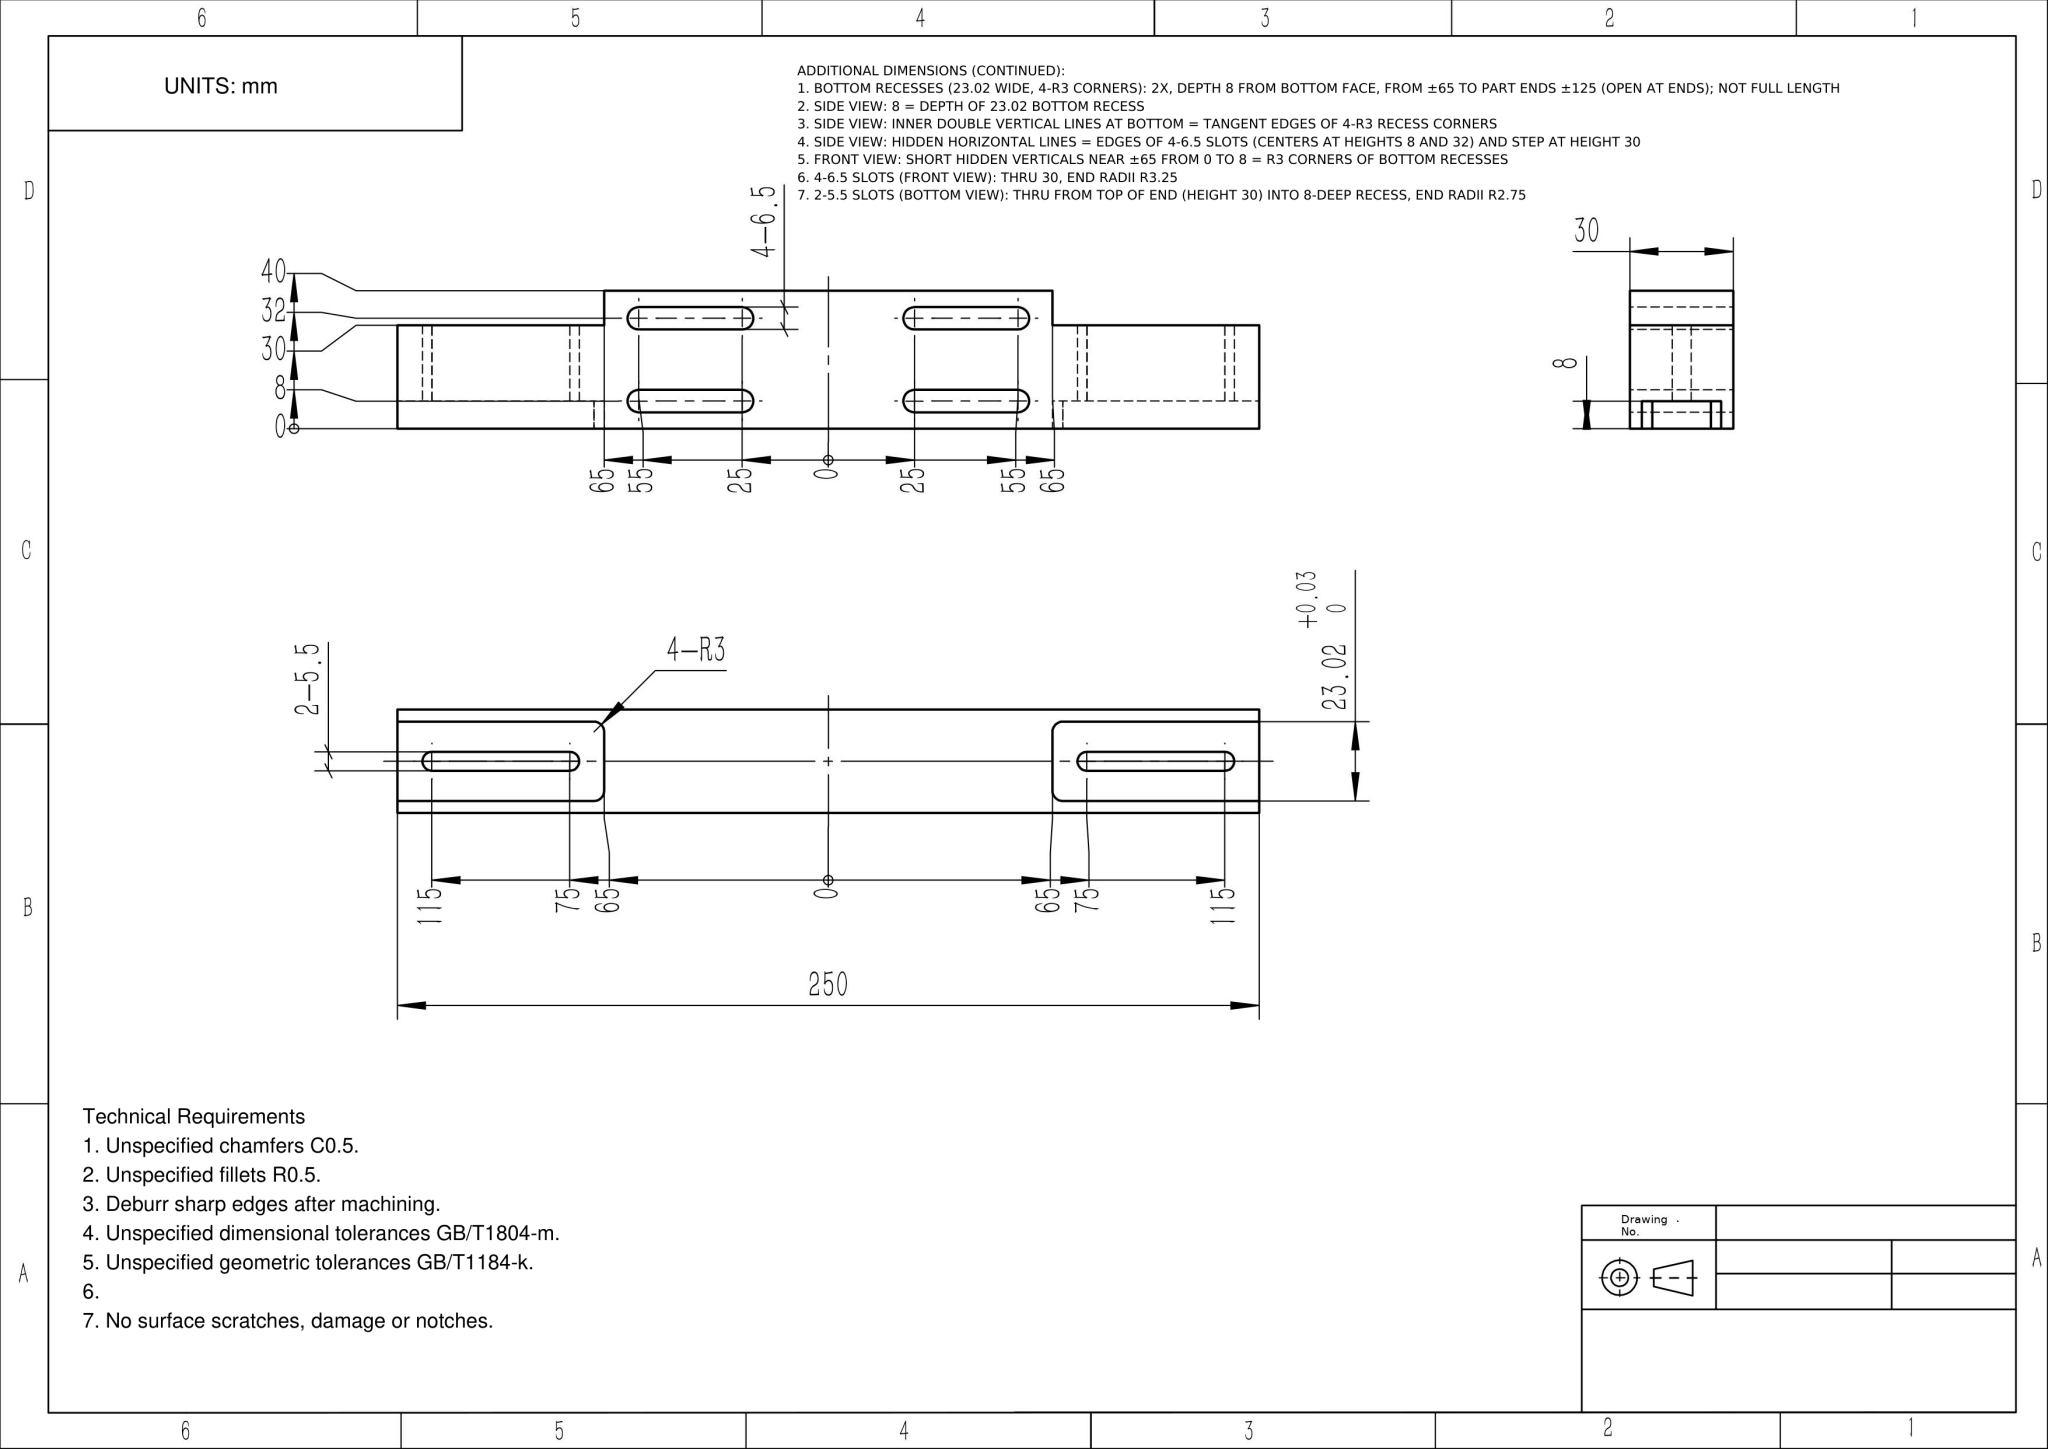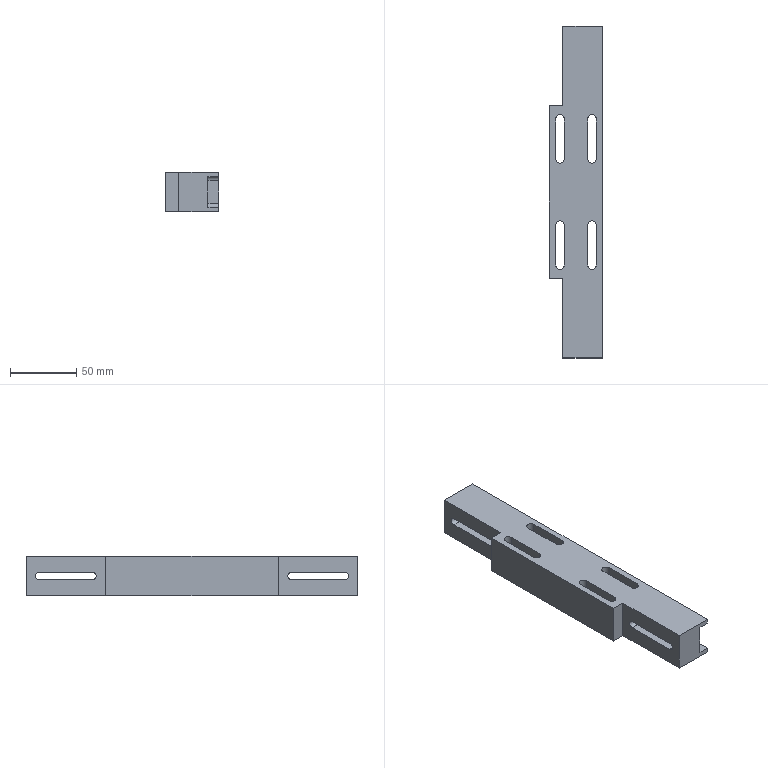Part | NX | mm | 1 solid | 46 faces | box 40 x 250 x 30 mm | volume 203855 mm3 | plane 30 | cylinder 16 | commonest cylinder face diameters 6.5 x8 5.5 x4 6 x4